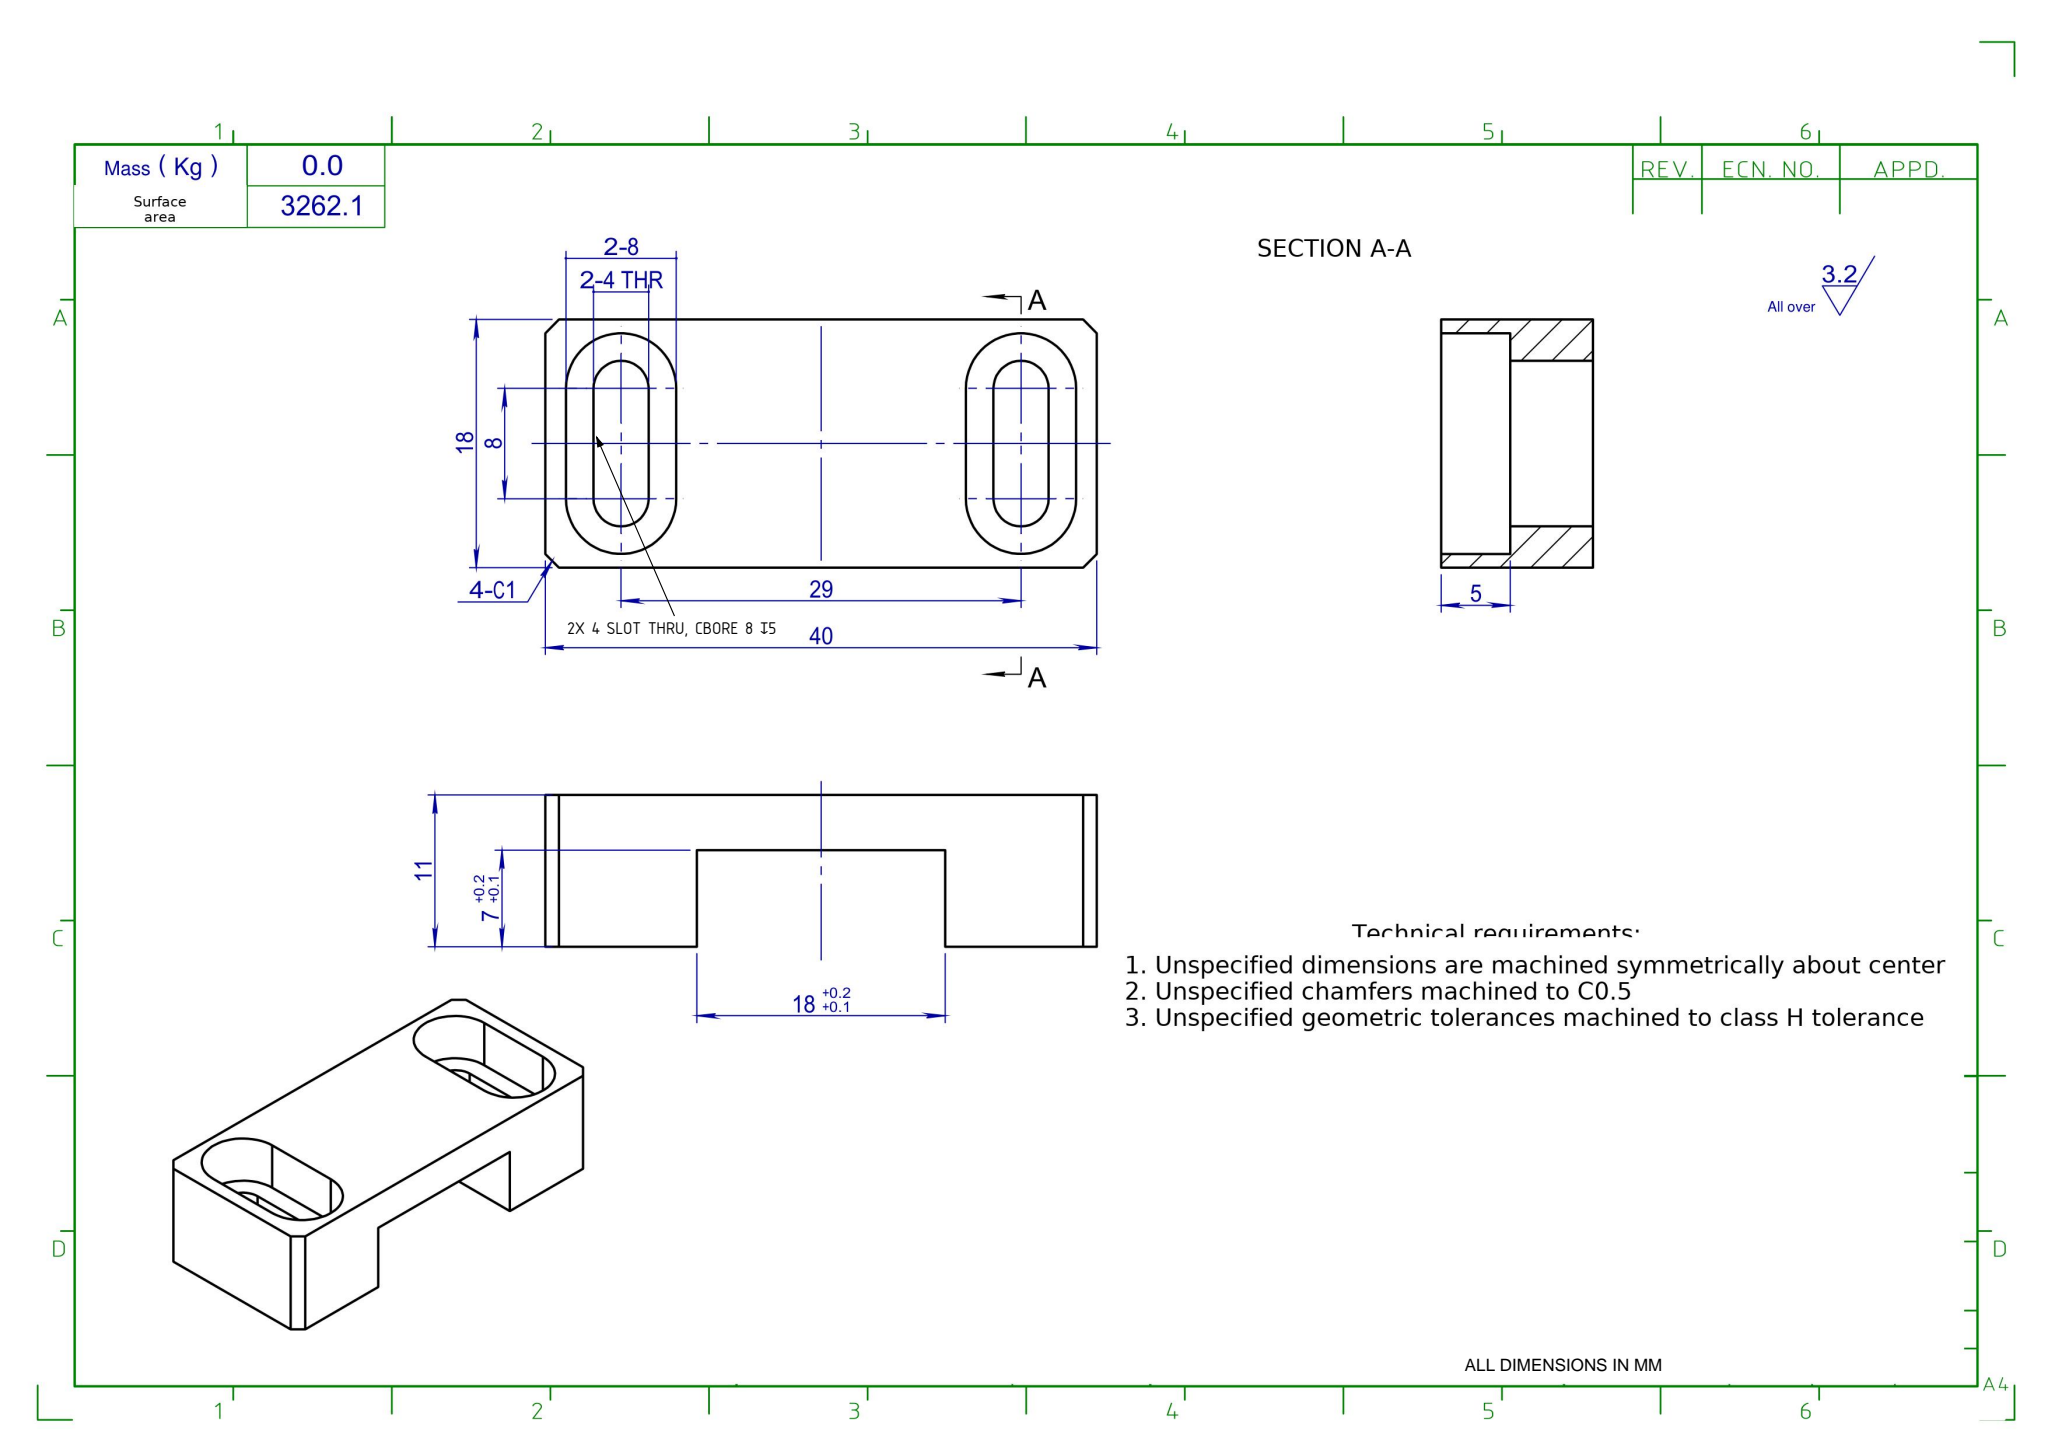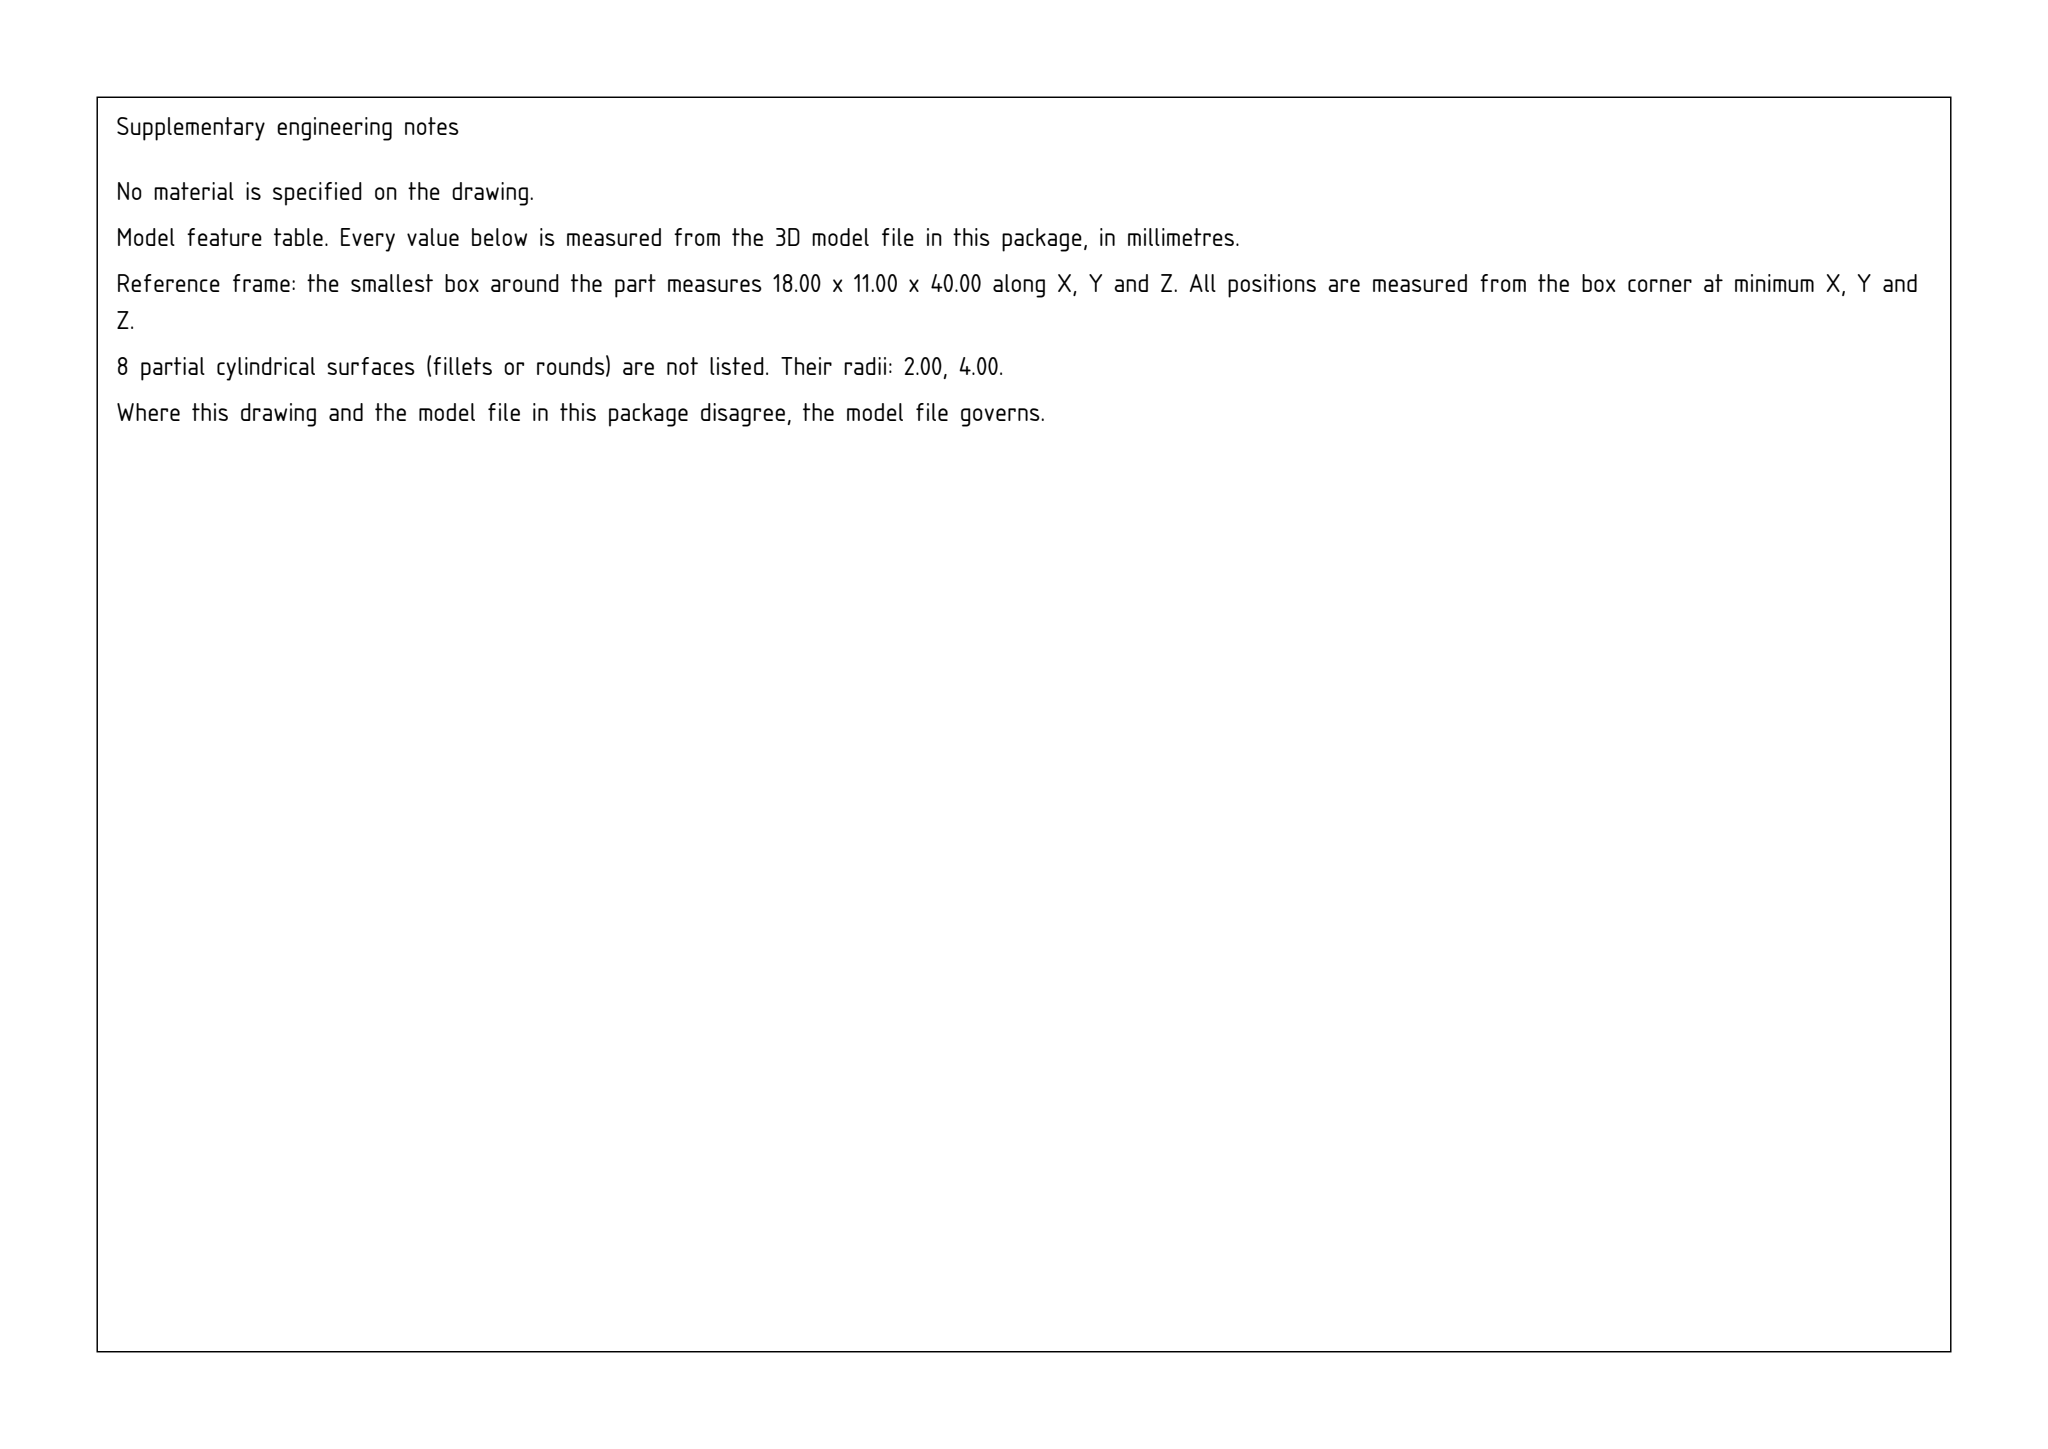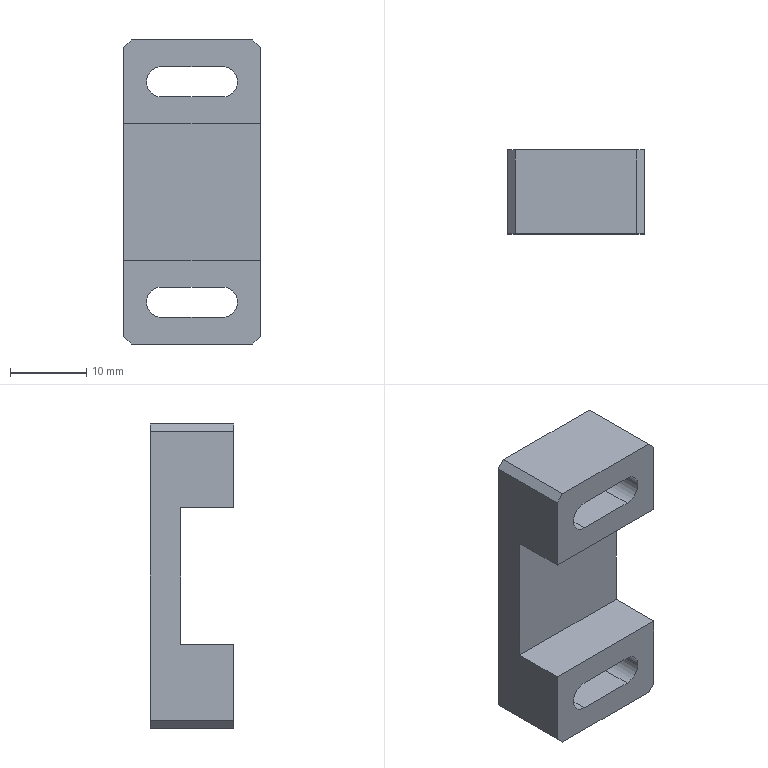Part | SolidWorks | mm | 1 solid | 32 faces | box 18 x 11 x 40 mm | volume 3953 mm3 | plane 24 | cylinder 8 | commonest cylinder face diameters 4 x4 8 x4
Drawing notes:
2-4 THR: 2X SLOT 4 WIDE THRU, CTRS 8 APART; C'BORE 8 WIDE DP 5 | from the solid: Ø4 half-arcs at x=5 & 13 (8 apart), z=5.5 & 34.5, y 0-6 thru; Ø8 half-arcs same centers y 6-11 (5 deep)
build123d program:
from build123d import *

# Parameters (mm, degrees)
SKETCH1_W          = 18
SKETCH1_H          = 40
EXTRUDE1_DEPTH     = 11
SKETCH2_W          = 18
SKETCH2_H          = 18
CUT_EXTRUDE1_DEPTH = 7
CUT_EXTRUDE2_DEPTH = 25.536
CUT_EXTRUDE3_DEPTH = 5
CHAMFER1_SIZE      = 1


with BuildPart() as part:
    # Sketch1 → Extrude1 (new body)
    with BuildSketch(Plane(origin=(0, 0, 0), x_dir=(1, 0, 0), z_dir=(0, 1, 0))):
        Rectangle(SKETCH1_W, SKETCH1_H)
    extrude(amount=EXTRUDE1_DEPTH)

    # Sketch2 → Cut-Extrude1 (cut)
    with BuildSketch(Plane.XZ):
        Rectangle(SKETCH2_W, SKETCH2_H)
    extrude(amount=-CUT_EXTRUDE1_DEPTH, mode=Mode.SUBTRACT)

    # Sketch3 → Cut-Extrude2 (cut, through all)
    with BuildSketch(Plane(origin=(0, 11, 0), x_dir=(1, 0, 0), z_dir=(0, 1, 0))):
        with BuildLine():
            Line((-4, 12.5), (4, 12.5))
            ThreePointArc((4, 12.5), (6, 14.5), (4, 16.5))
            Line((4, 16.5), (-4, 16.5))
            ThreePointArc((-4, 16.5), (-6, 14.5), (-4, 12.5))
        make_face()
        with BuildLine():
            Line((-4, -16.5), (4, -16.5))
            ThreePointArc((4, -16.5), (6, -14.5), (4, -12.5))
            Line((4, -12.5), (-4, -12.5))
            ThreePointArc((-4, -12.5), (-6, -14.5), (-4, -16.5))
        make_face()
    extrude(amount=-CUT_EXTRUDE2_DEPTH, mode=Mode.SUBTRACT)

    # Sketch4 → Cut-Extrude3 (cut)
    with BuildSketch(Plane(origin=(0, 11, 0), x_dir=(1, 0, 0), z_dir=(0, 1, 0))):
        with BuildLine():
            Line((-4, -18.5), (4, -18.5))
            ThreePointArc((4, -18.5), (8, -14.5), (4, -10.5))
            Line((4, -10.5), (-4, -10.5))
            ThreePointArc((-4, -10.5), (-8, -14.5), (-4, -18.5))
        make_face()
        with BuildLine():
            Line((4, 10.5), (-4, 10.5))
            ThreePointArc((-4, 10.5), (-8, 14.5), (-4, 18.5))
            Line((-4, 18.5), (4, 18.5))
            ThreePointArc((4, 18.5), (8, 14.5), (4, 10.5))
        make_face()
    extrude(amount=-CUT_EXTRUDE3_DEPTH, mode=Mode.SUBTRACT)

    # Chamfer1
    chamfer1_edges = [part.edges().sort_by_distance(p)[0] for p in [
        (-9, 5.5, -20),
        (9, 5.5, -20),
        (9, 5.5, 20),
        (-9, 5.5, 20),
    ]]
    chamfer(chamfer1_edges, length=CHAMFER1_SIZE)


solid = part.part